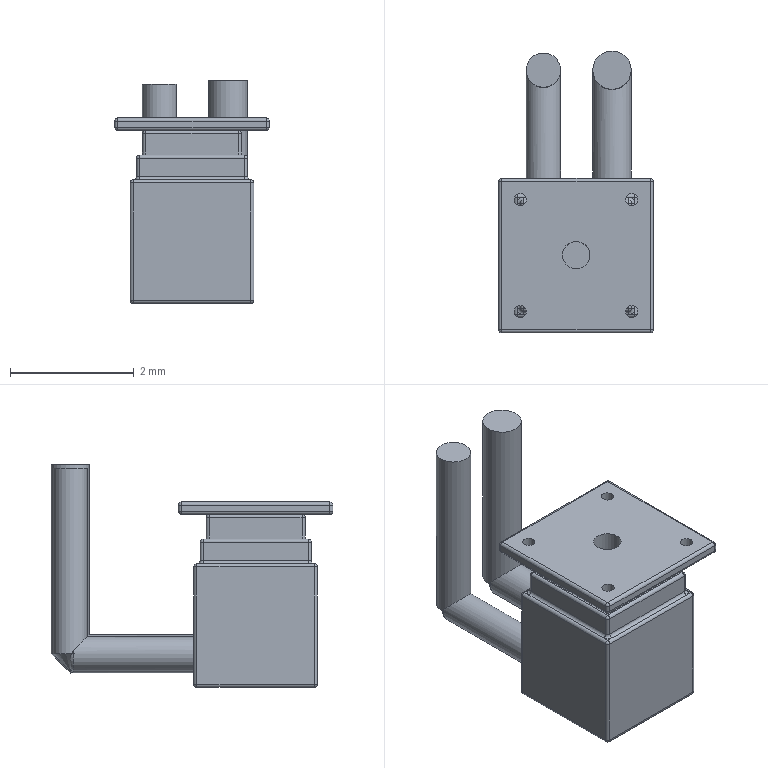Component | NX | H2 | 5 solids | 122 faces | volume 14 mm3 | cylinder 55 | plane 33 | sphere 24 | torus 6 | cone 4 | commonest cylinder face diameters 0.1 x44 0.2 x4 0.555 x3 0.622 x3 0.442 x1